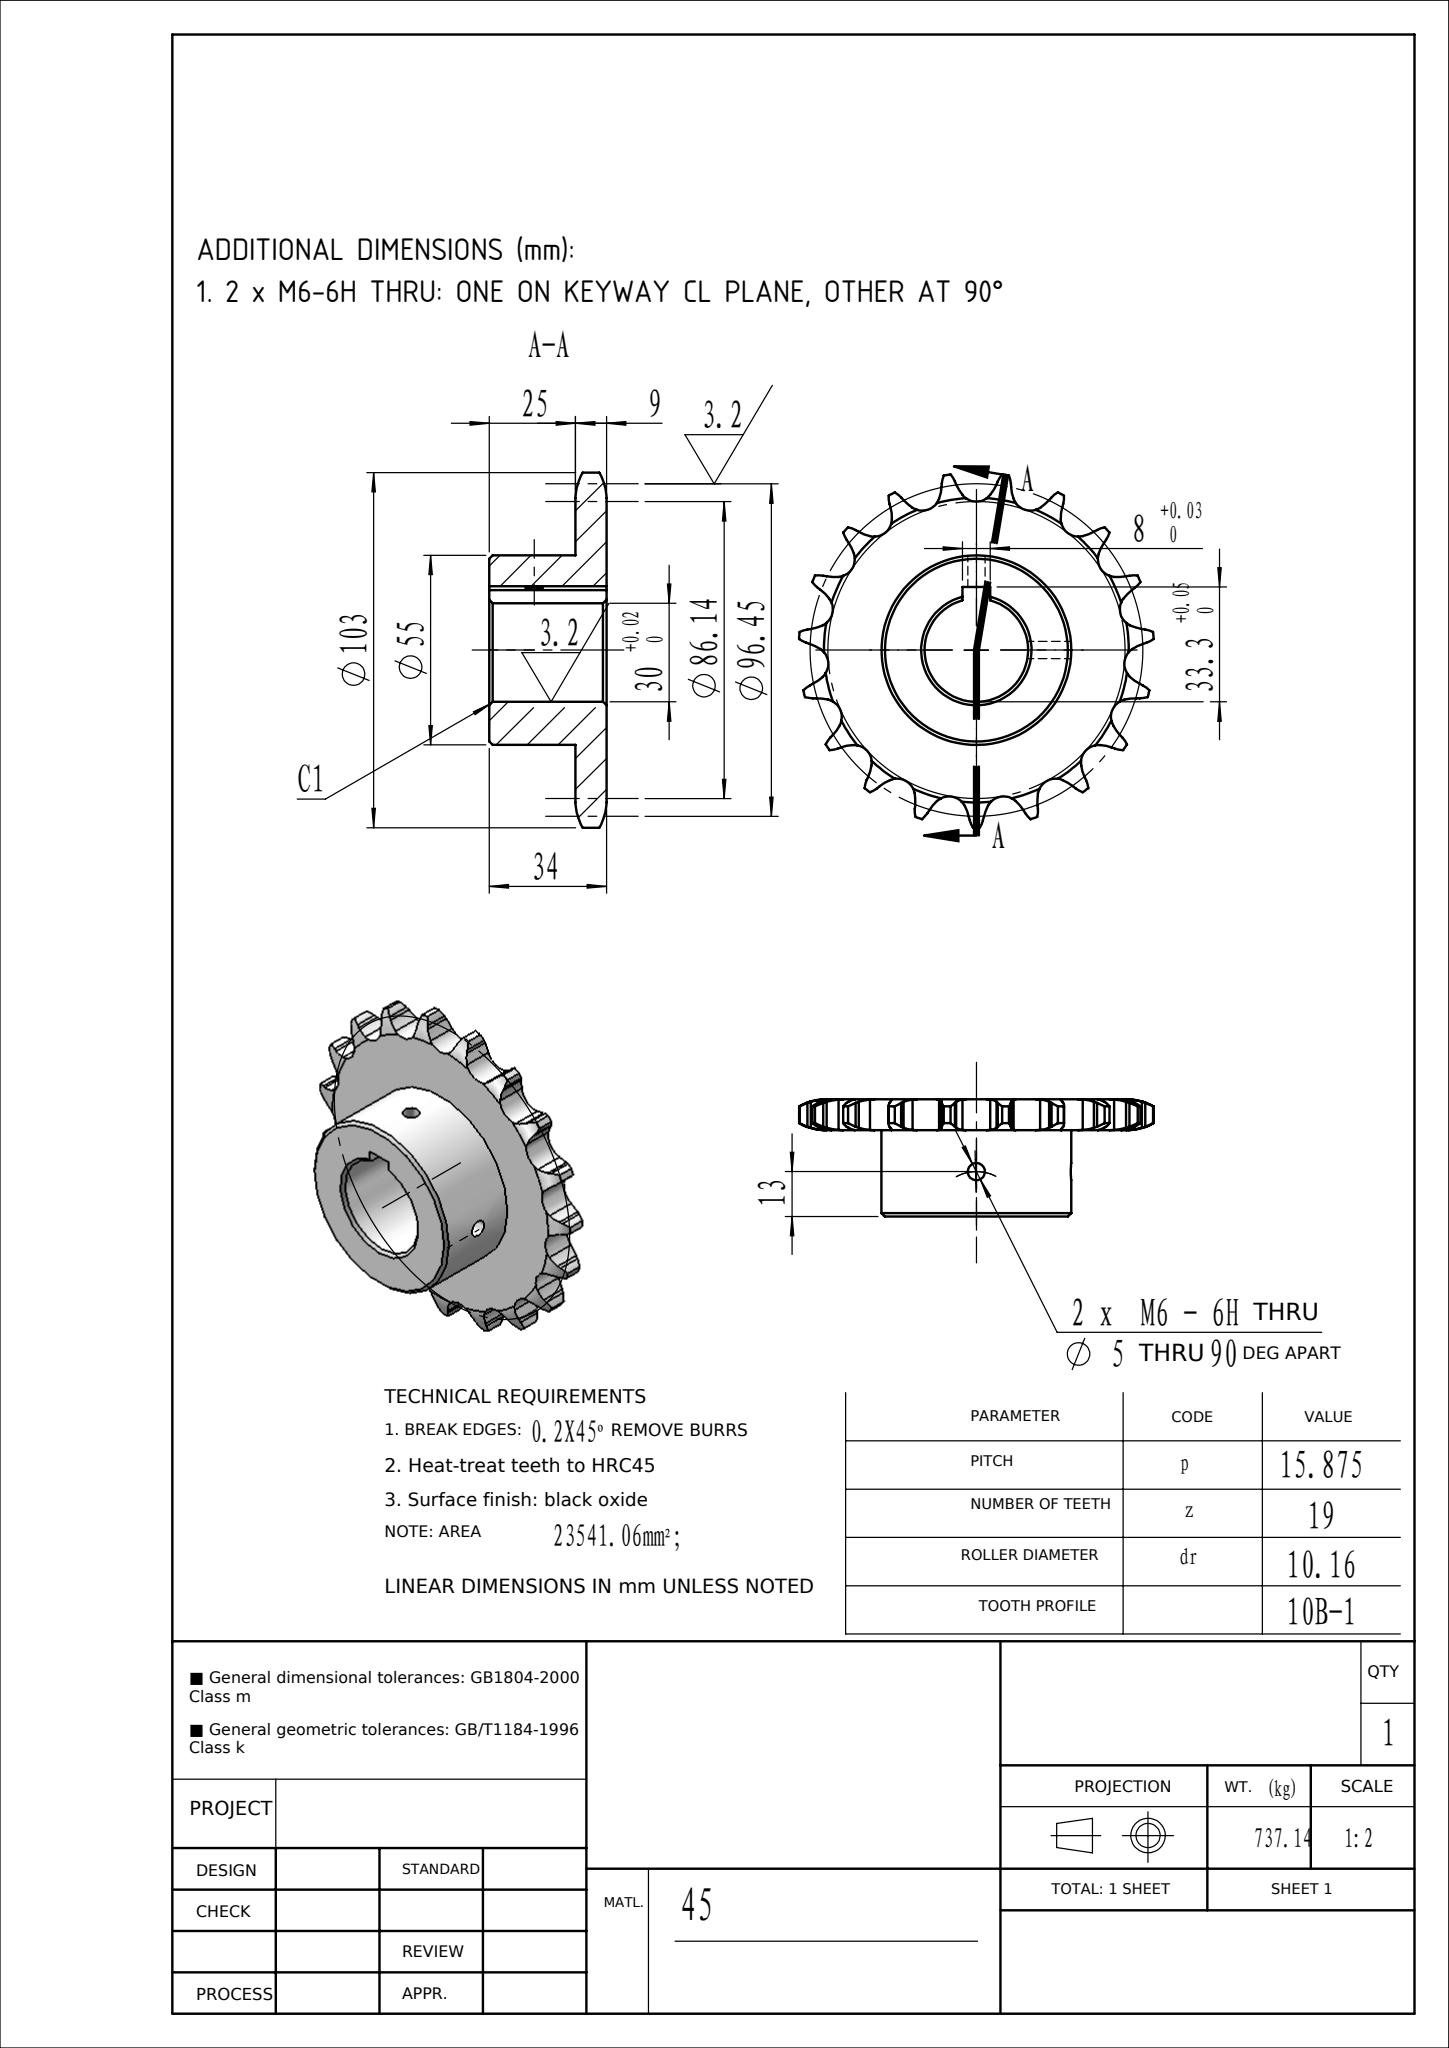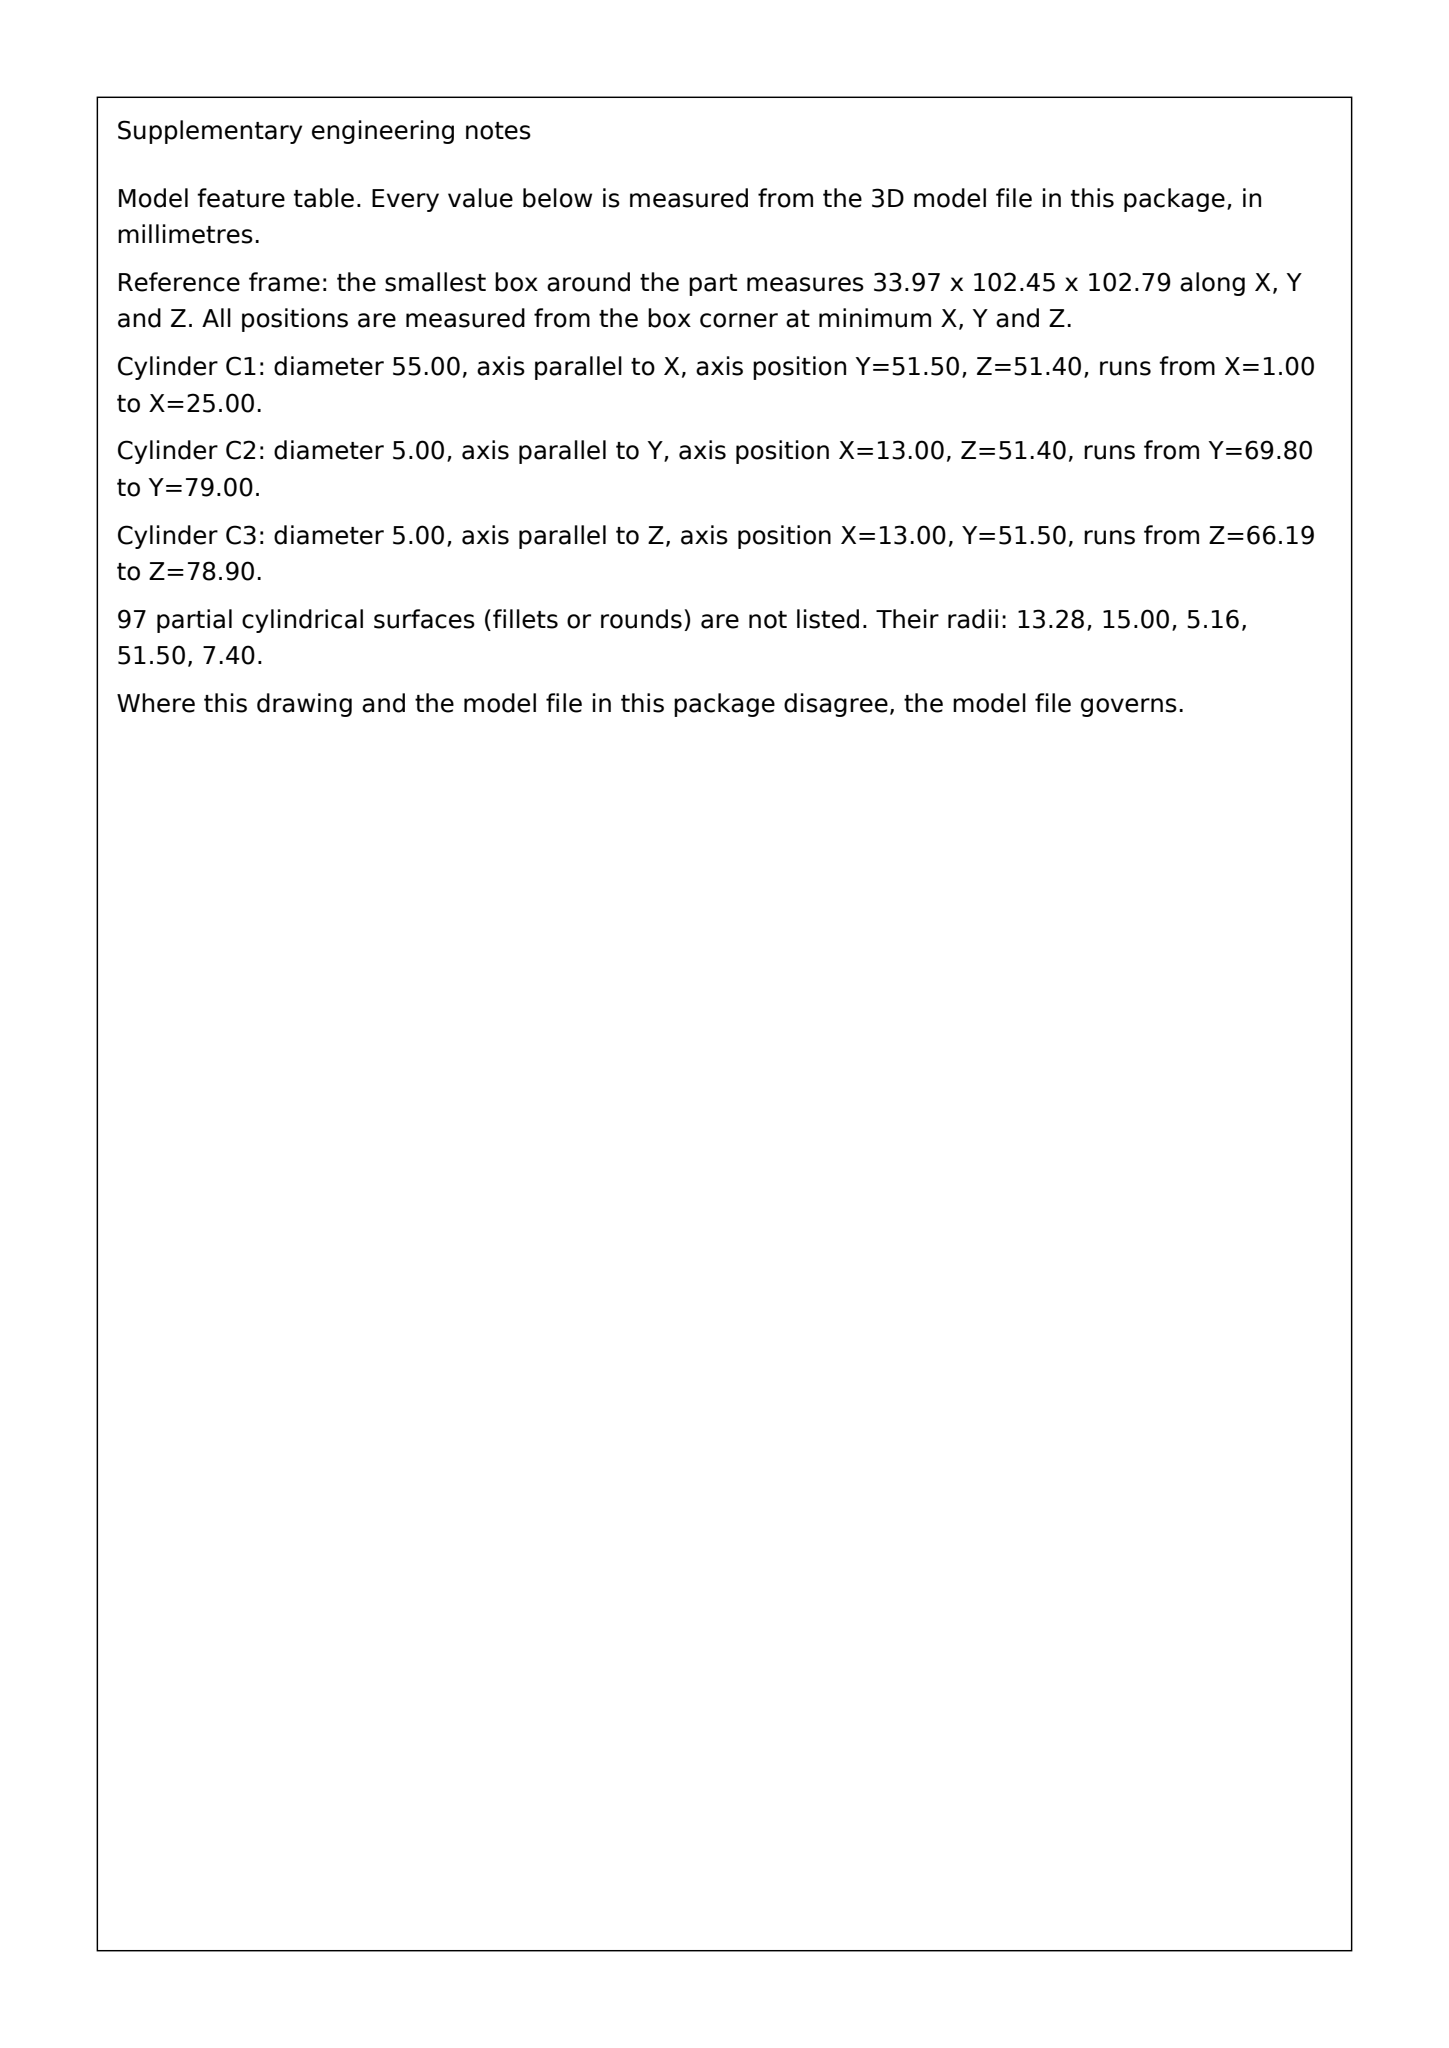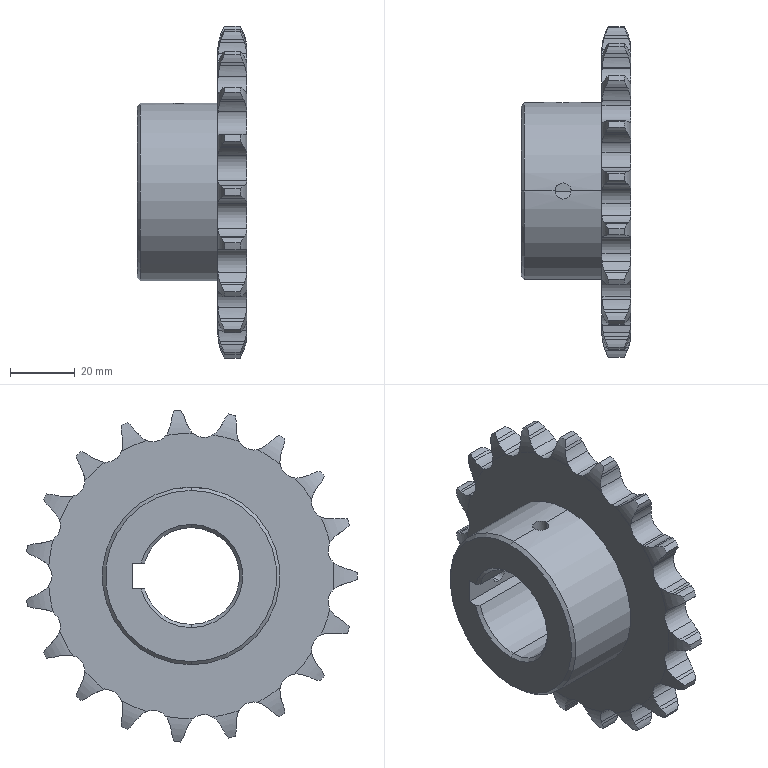Part | SolidWorks | mm | 1 solid | 224 faces | box 33.97 x 102.45 x 102.79 mm | volume 93428 mm3 | cylinder 132 | plane 44 | torus 40 | cone 8 | commonest cylinder face diameters 14.803 x40 26.567 x40 10.311 x24 103 x19 5 x4 30 x3 55 x2